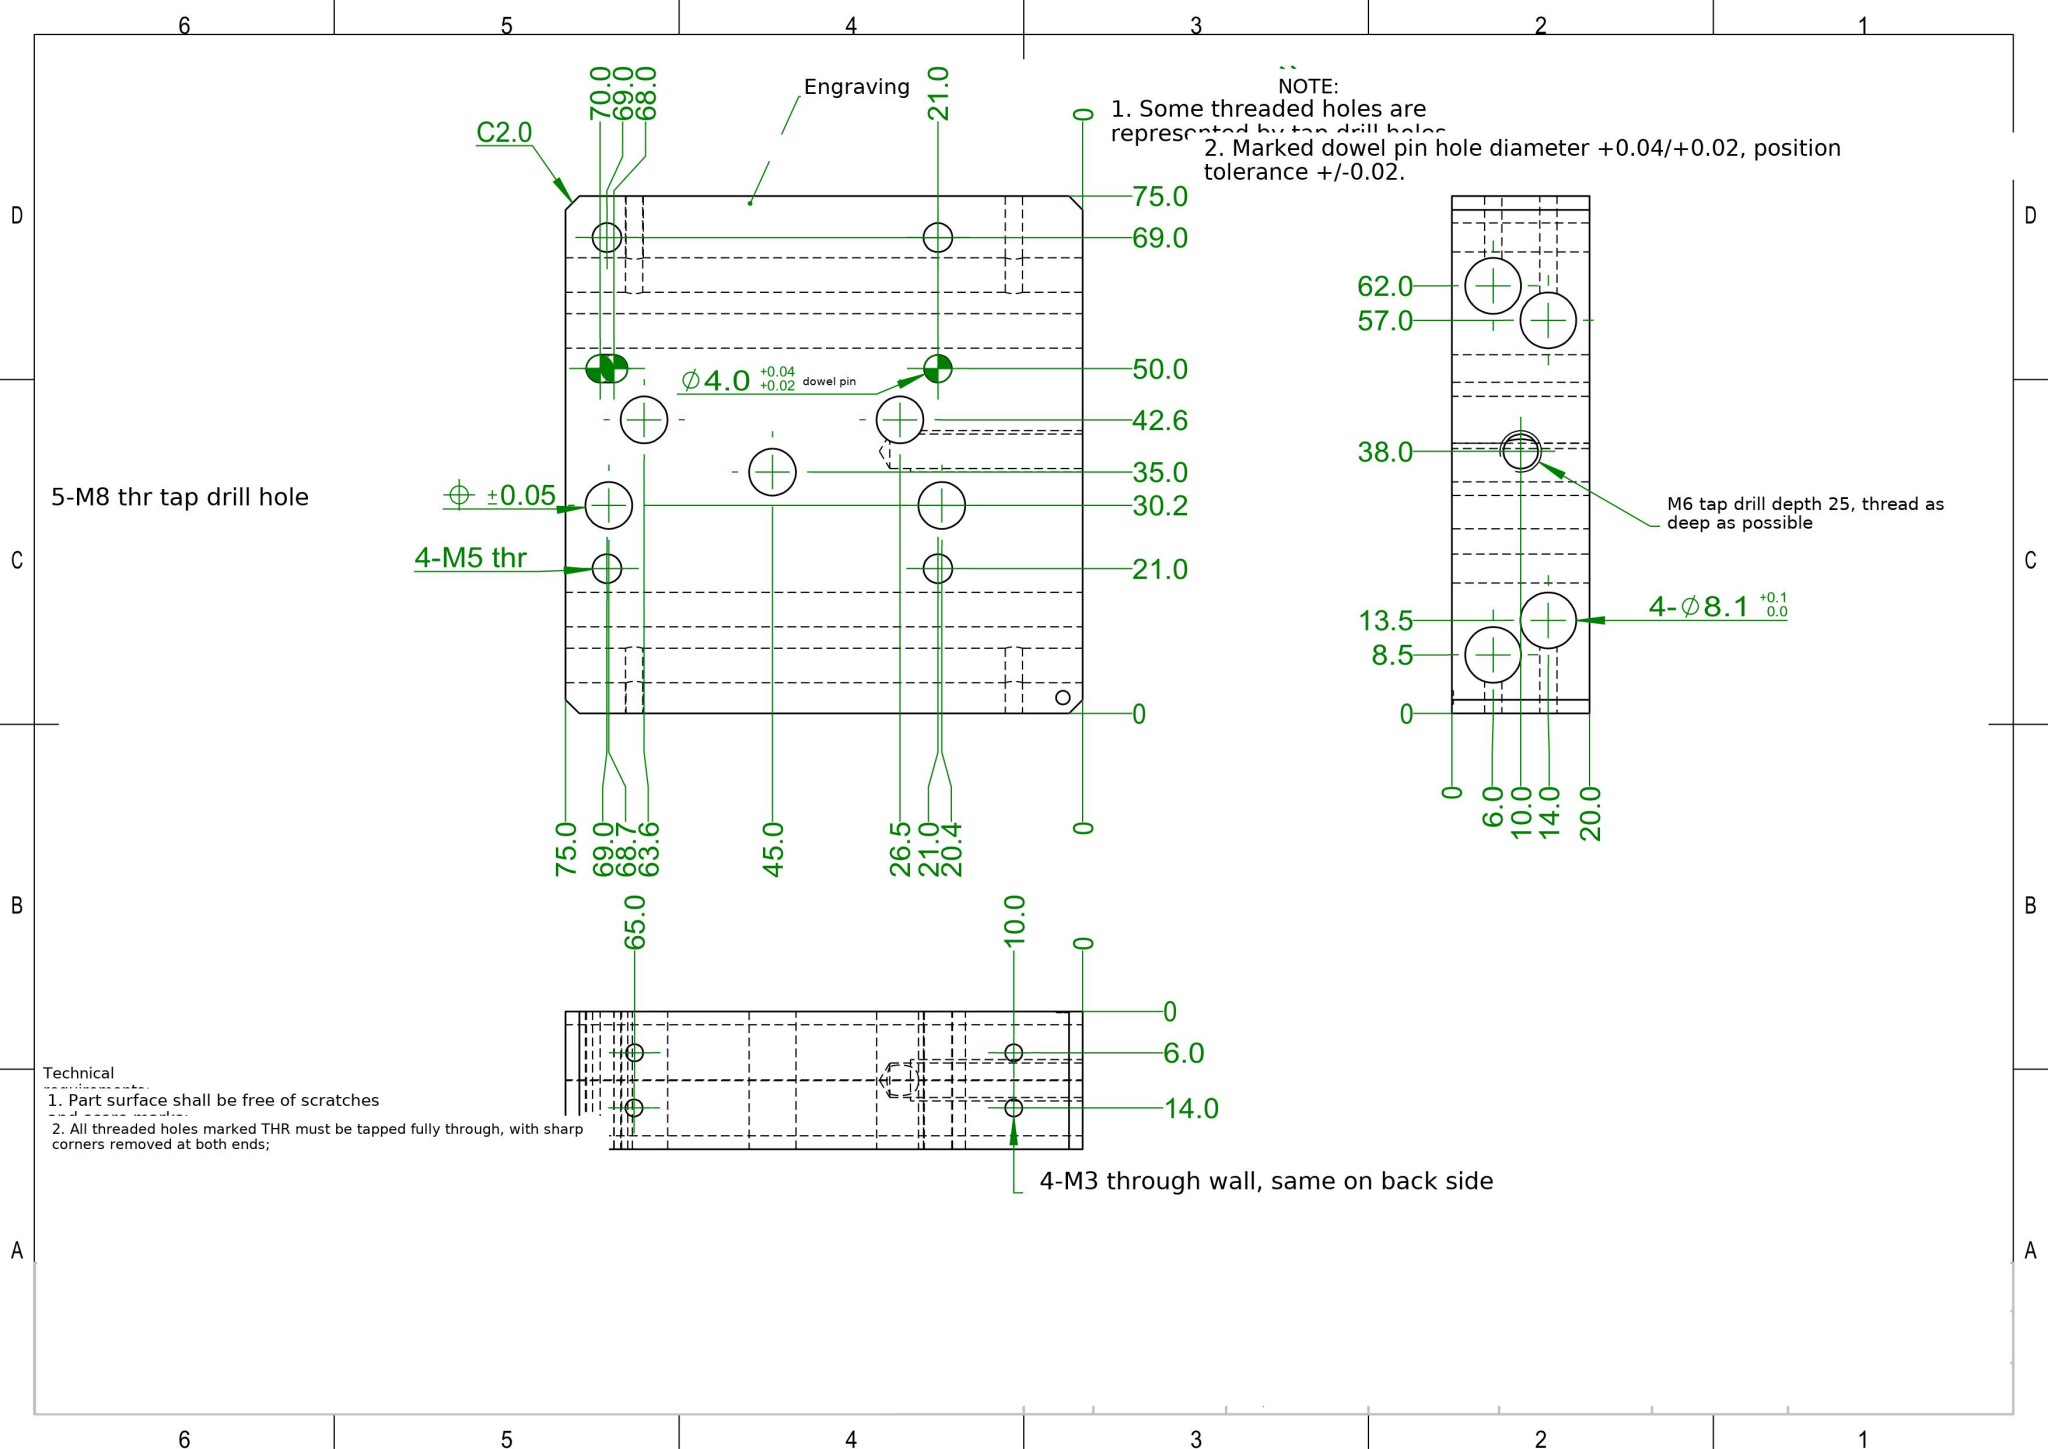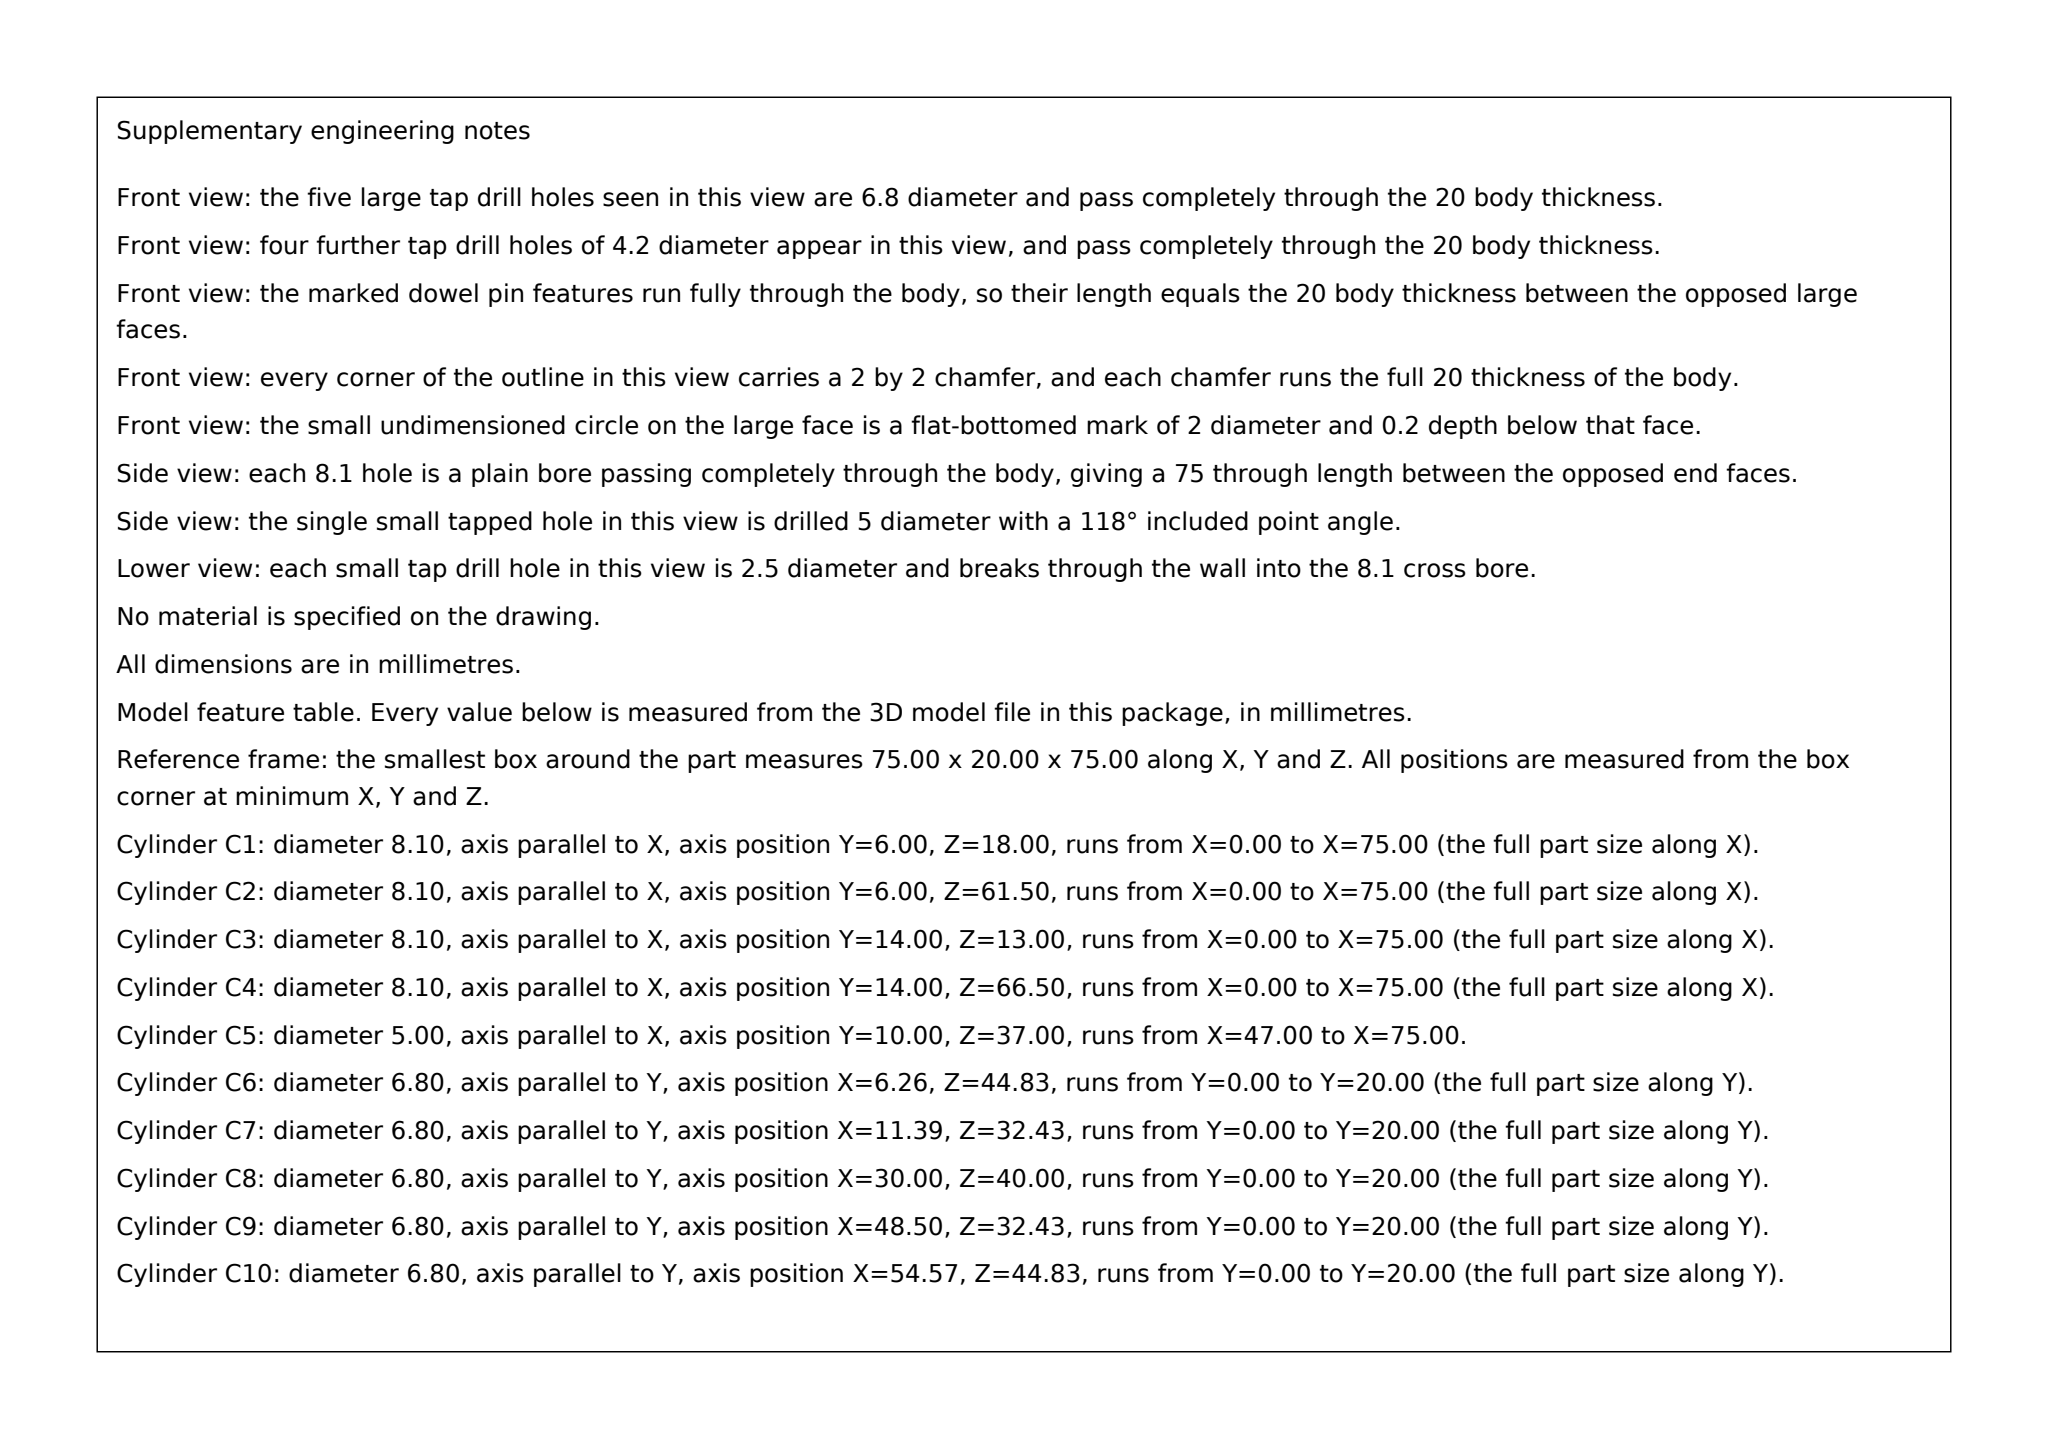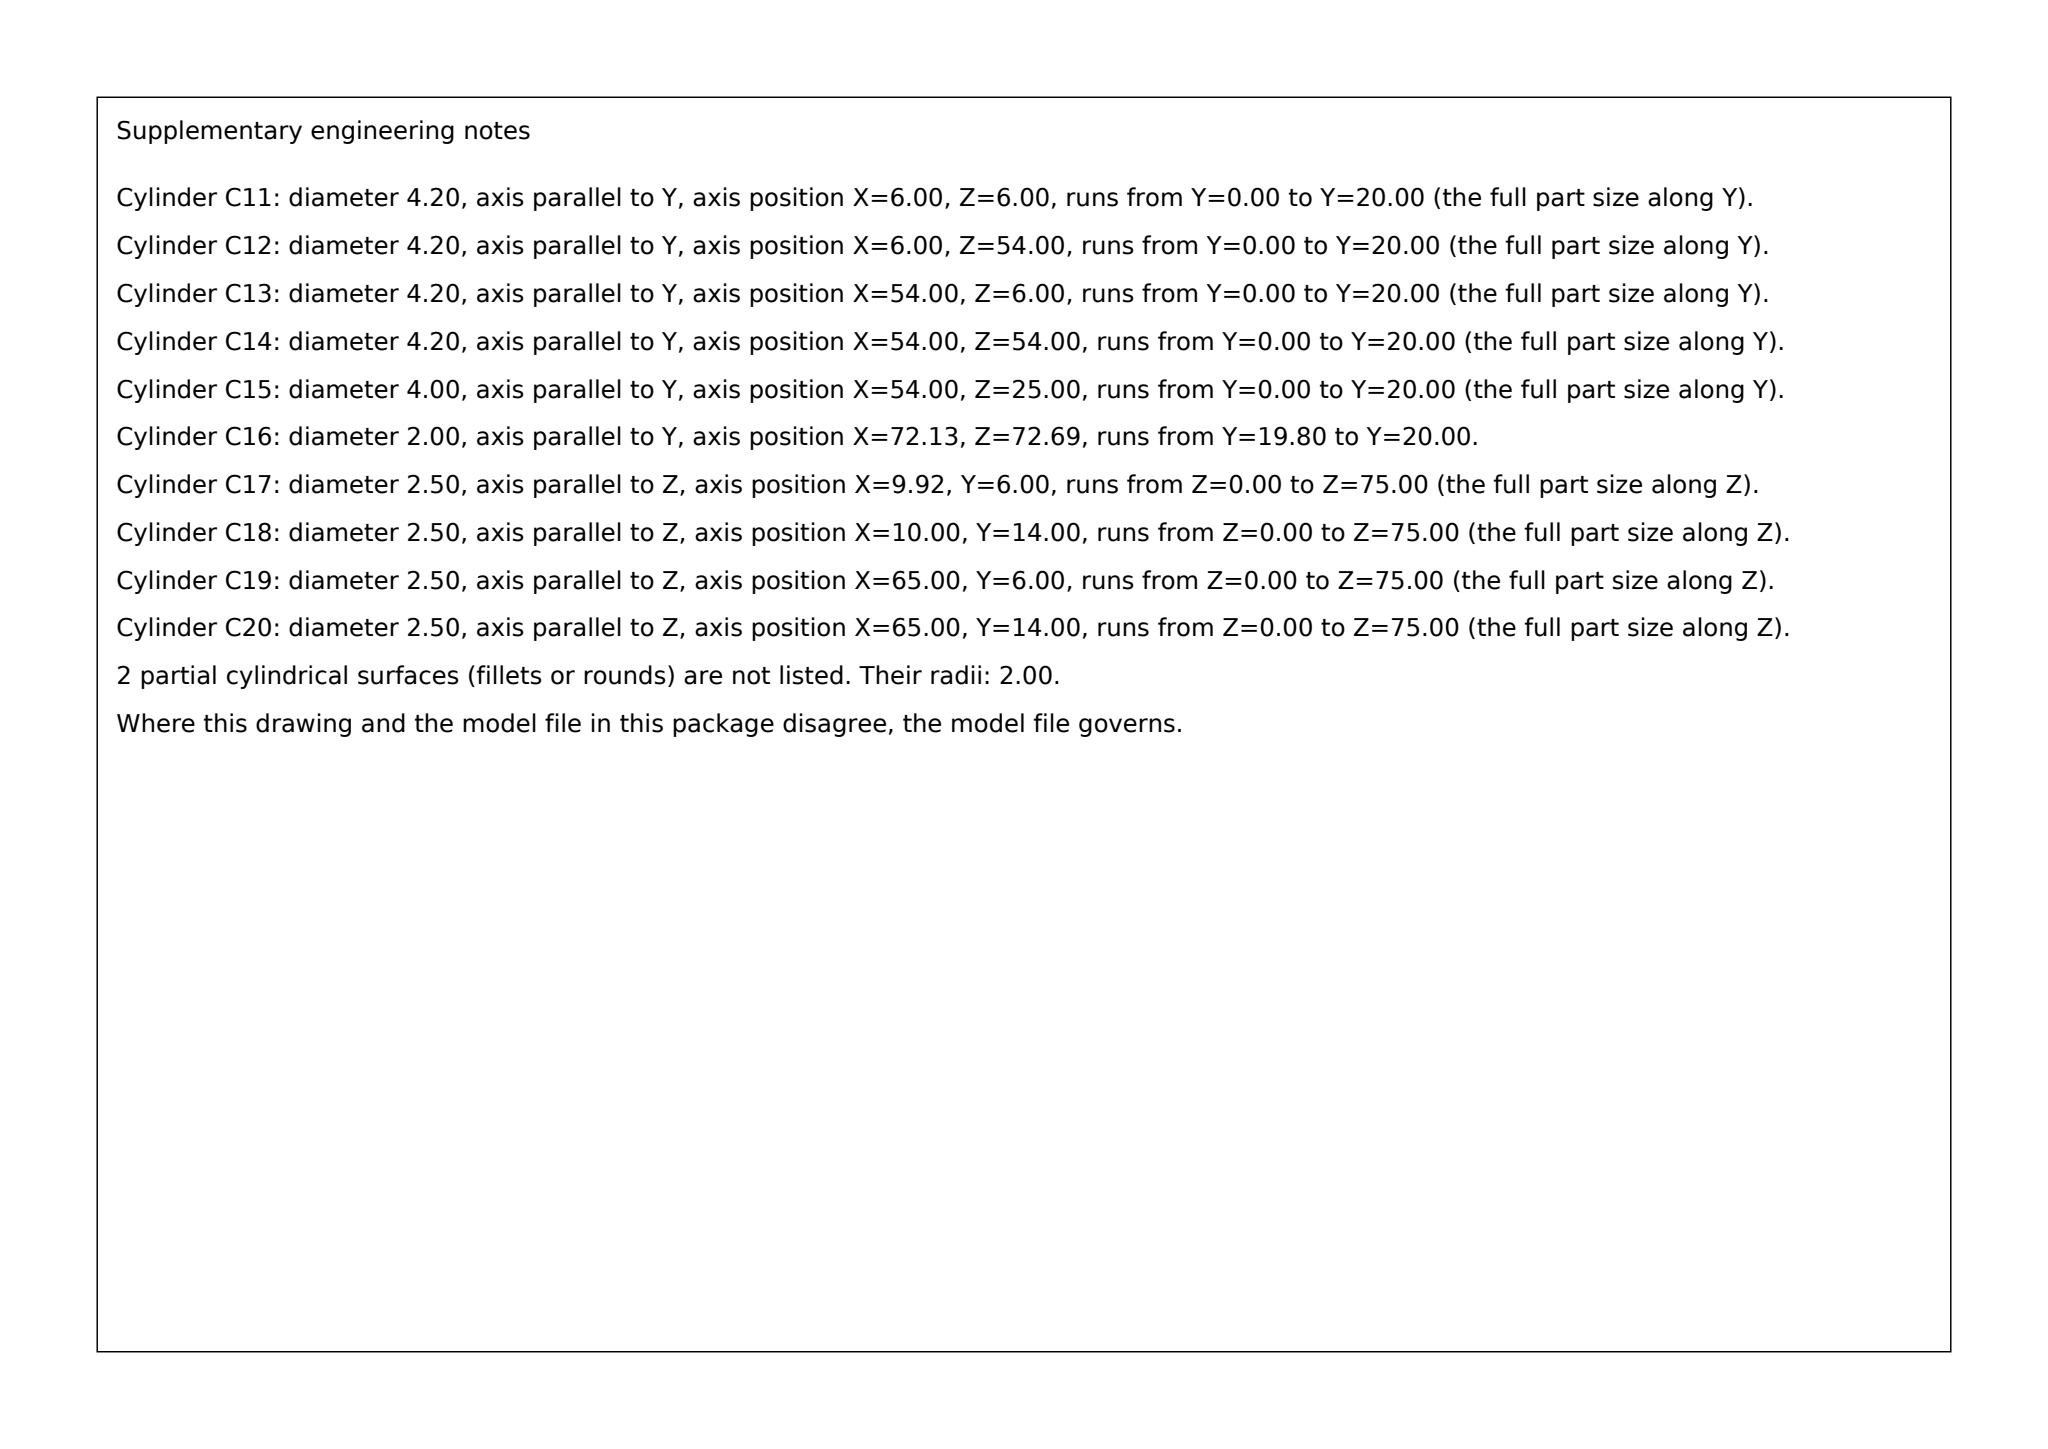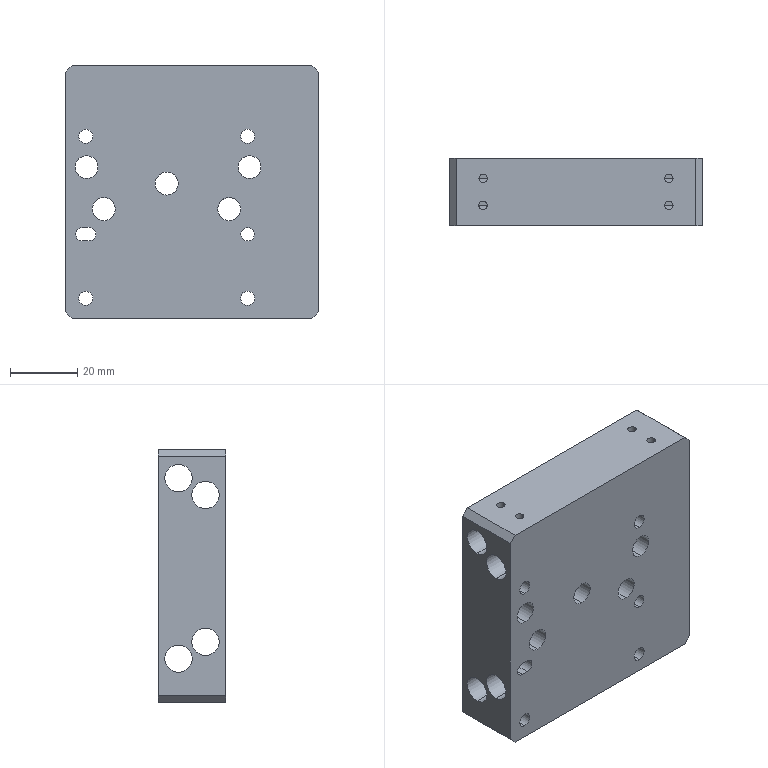Part | SolidWorks | mm | 1 solid | 65 faces | box 75 x 20 x 75 mm | volume 90568 mm3 | cylinder 50 | plane 13 | cone 2 | commonest cylinder face diameters 2.5 x16 6.8 x10 8.1 x8 4.2 x8 4 x4 5 x2 2 x2
Drawing notes:
Ø2.0 DP 0.2 MARK HOLE 2.87 FROM RH EDGE, 2.31 FROM BTM, 2X BOTH FACES | from the solid: cyl dia2.0 axis y at x=72.13,z=72.69, len 0.2, count 2; bbox 75x20x75 -> 75-72.13=2.87, 75-72.69=2.31; y planes 0 & 19.8
4-M5 TAP THRU 20; Ø4.2 TAP DRILL THRU | from the solid: 4 cyl dia4.2 (M5 tap drill) axis y, length 20 thru, at x/z = 6/6, 6/54, 54/6, 54/54
5-M8 THR: Ø6.8 BOTTOM HOLE THRU 20 THK | from the solid: 5 cyl Ø6.8 axis y, len 20.0 = full 20 thickness (6.26/44.83, 11.39/32.43, 30/40, 48.5/32.43, 54.57/44.83)
DOWEL SLOT: 4.0 WIDE x 6.0 LG THRU, CTRS AT 70.0 & 68.0 | from the solid: two Ø4.0 axis y bores at x=5.0 and x=7.0, z=25, len 20 -> 2.0 ctr spacing, 4 wide x 6 long slot; 75-5=70.0, 75-7=68.0
4-Ø8.1 +0.1/0.0 THRU, 75 LG | from the solid: cyl dia 8.1 axis x length 75.0 (=bbox x) at y6/z18, y6/z61.5, y14/z13, y14/z66.5
2X M6: Ø5.0 DRILL DP 28, 1 EACH END FACE, 37.0 FROM BTM | from the solid: cyl dia 5.0 axis x, pos y10.0 z37.0, length 28.0, count 2 (one per end face x=0 / x=75)
M6 THD DP 25 FULL AFTER Ø5.0 DRILL DP 28, 118° PT, 2 PLCS | from the solid: dia 5.0 drill 28 deep, cone 118° ref dia 5.0, count 2
4-M3 THRU WALL (Ø2.5 DRILL), SAME 4 ON BACK = 8 PLCS | from the solid: dia 2.5 axis z at x10/65, y6/14, segments 4.65-14.15 lg, count 2 each (both faces)
2X Ø2.0 DP 0.2 MARK HOLE BOTH FACES: 2.87 FROM RH, 2.31 FROM BTM | from the solid: dia 2.0 axis y, pos x72.13 z72.69, length 0.2, count 2 (y=0 and y=19.8 faces)